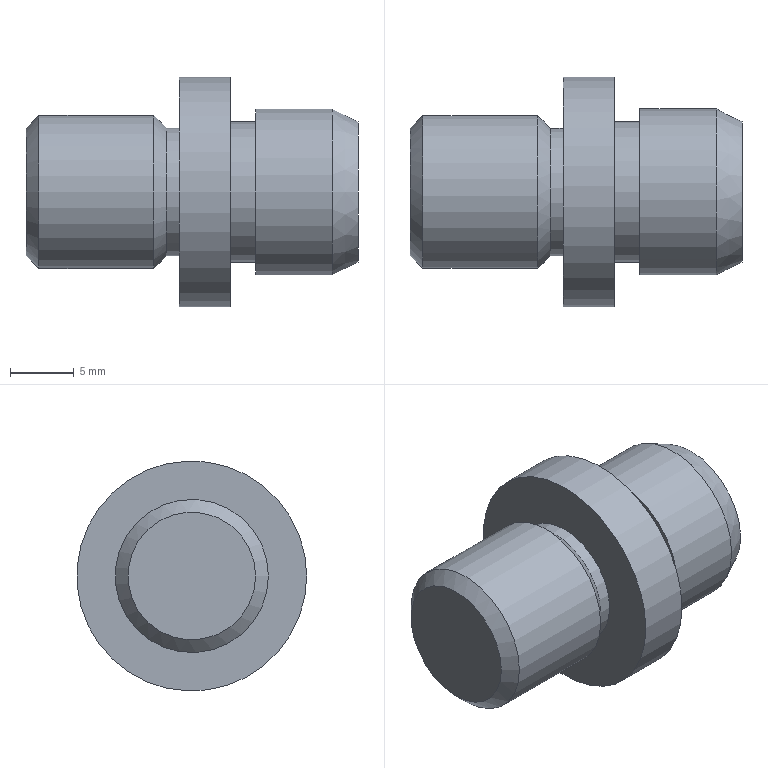Component | NX | LOC_PIN | 1 solid | 13 faces | box 26 x 18 x 18 mm | volume 3518 mm3 | plane 5 | cylinder 5 | cone 3 | commonest cylinder face diameters 12 x1 10 x1 18 x1 11 x1 13 x1
STEP:
#1=CARTESIAN_POINT('',(0.,0.,0.));
#2=DIRECTION('',(0.,0.,1.));
#3=DIRECTION('',(1.,0.,0.));
#4=AXIS2_PLACEMENT_3D('',#1,#2,#3);
#5=CARTESIAN_POINT('',(6.,75.339,-338.901));
#6=VERTEX_POINT('',#5);
#7=CARTESIAN_POINT('',(6.,80.839,-338.901));
#8=DIRECTION('',(-1.,-0.,0.));
#9=DIRECTION('',(0.,-1.,0.));
#10=AXIS2_PLACEMENT_3D('',#7,#8,#9);
#11=CIRCLE('',#10,5.5);
#12=CARTESIAN_POINT('',(6.,80.839,-338.901));
#13=DIRECTION('',(-1.,-0.,0.));
#14=DIRECTION('',(0.,-1.,0.));
#15=AXIS2_PLACEMENT_3D('',#12,#13,#14);
#16=PLANE('',#15);
#17=CARTESIAN_POINT('',(0.,0.));
#18=DIRECTION('',(1.,0.));
#19=AXIS2_PLACEMENT_2D('',#17,#18);
#20=CIRCLE('',#19,5.5);
#21=(GEOMETRIC_REPRESENTATION_CONTEXT(2)PARAMETRIC_REPRESENTATION_CONTEXT()REPRESENTATION_CONTEXT('',''));
#22=DEFINITIONAL_REPRESENTATION('',(#20),#21);
#23=PCURVE('',#16,#22);
#24=CARTESIAN_POINT('',(6.,80.839,-338.901));
#25=DIRECTION('',(-1.,-0.,0.));
#26=DIRECTION('',(0.,-1.,0.));
#27=AXIS2_PLACEMENT_3D('',#24,#25,#26);
#28=CONICAL_SURFACE('',#27,5.5,0.4636);
#29=CARTESIAN_POINT('',(0.,0.));
#30=DIRECTION('',(1.,0.));
#31=VECTOR('',#30,1.);
#32=LINE('',#29,#31);
#33=(GEOMETRIC_REPRESENTATION_CONTEXT(2)PARAMETRIC_REPRESENTATION_CONTEXT()REPRESENTATION_CONTEXT('',''));
#34=DEFINITIONAL_REPRESENTATION('',(#32),#33);
#35=PCURVE('',#28,#34);
#36=SURFACE_CURVE('',#11,(#23,#35),.PCURVE_S1.);
#37=EDGE_CURVE('',#6,#6,#36,.T.);
#38=ORIENTED_EDGE('',*,*,#37,.F.);
#39=EDGE_LOOP('',(#38));
#40=FACE_BOUND('',#39,.T.);
#41=ADVANCED_FACE('',(#40),#16,.F.);
#42=CARTESIAN_POINT('',(-20.,75.839,-338.901));
#43=VERTEX_POINT('',#42);
#44=CARTESIAN_POINT('',(-20.,80.839,-338.901));
#45=DIRECTION('',(-1.,-0.,0.));
#46=DIRECTION('',(0.,-1.,0.));
#47=AXIS2_PLACEMENT_3D('',#44,#45,#46);
#48=CIRCLE('',#47,5.);
#49=CARTESIAN_POINT('',(-20.,80.839,-338.901));
#50=DIRECTION('',(-1.,-0.,0.));
#51=DIRECTION('',(0.,-1.,0.));
#52=AXIS2_PLACEMENT_3D('',#49,#50,#51);
#53=PLANE('',#52);
#54=CARTESIAN_POINT('',(0.,0.));
#55=DIRECTION('',(1.,0.));
#56=AXIS2_PLACEMENT_2D('',#54,#55);
#57=CIRCLE('',#56,5.);
#58=(GEOMETRIC_REPRESENTATION_CONTEXT(2)PARAMETRIC_REPRESENTATION_CONTEXT()REPRESENTATION_CONTEXT('',''));
#59=DEFINITIONAL_REPRESENTATION('',(#57),#58);
#60=PCURVE('',#53,#59);
#61=CARTESIAN_POINT('',(-19.,80.839,-338.901));
#62=DIRECTION('',(1.,0.,0.));
#63=DIRECTION('',(-0.,1.,0.));
#64=AXIS2_PLACEMENT_3D('',#61,#62,#63);
#65=CONICAL_SURFACE('',#64,6.,0.7854);
#66=CARTESIAN_POINT('',(9.425,-1.));
#67=DIRECTION('',(-1.,0.));
#68=VECTOR('',#67,1.);
#69=LINE('',#66,#68);
#70=(GEOMETRIC_REPRESENTATION_CONTEXT(2)PARAMETRIC_REPRESENTATION_CONTEXT()REPRESENTATION_CONTEXT('',''));
#71=DEFINITIONAL_REPRESENTATION('',(#69),#70);
#72=PCURVE('',#65,#71);
#73=SURFACE_CURVE('',#48,(#60,#72),.PCURVE_S1.);
#74=EDGE_CURVE('',#43,#43,#73,.T.);
#75=ORIENTED_EDGE('',*,*,#74,.T.);
#76=EDGE_LOOP('',(#75));
#77=FACE_BOUND('',#76,.T.);
#78=ADVANCED_FACE('',(#77),#53,.T.);
#79=ORIENTED_EDGE('',*,*,#74,.F.);
#80=CARTESIAN_POINT('',(-19.,74.839,-338.901));
#81=VERTEX_POINT('',#80);
#82=CARTESIAN_POINT('',(-20.,75.839,-338.901));
#83=CARTESIAN_POINT('',(-19.,74.839,-338.901));
#84=B_SPLINE_CURVE_WITH_KNOTS('',1,(#82,#83),.UNSPECIFIED.,.F.,.F.,(2,2),(-1.414,-0.),.PIECEWISE_BEZIER_KNOTS.);
#85=CARTESIAN_POINT('',(9.425,0.));
#86=DIRECTION('',(0.,1.));
#87=VECTOR('',#86,1.);
#88=LINE('',#85,#87);
#89=(GEOMETRIC_REPRESENTATION_CONTEXT(2)PARAMETRIC_REPRESENTATION_CONTEXT()REPRESENTATION_CONTEXT('',''));
#90=DEFINITIONAL_REPRESENTATION('',(#88),#89);
#91=PCURVE('',#65,#90);
#92=CARTESIAN_POINT('',(3.142,0.));
#93=DIRECTION('',(0.,1.));
#94=VECTOR('',#93,1.);
#95=LINE('',#92,#94);
#96=(GEOMETRIC_REPRESENTATION_CONTEXT(2)PARAMETRIC_REPRESENTATION_CONTEXT()REPRESENTATION_CONTEXT('',''));
#97=DEFINITIONAL_REPRESENTATION('',(#95),#96);
#98=PCURVE('',#65,#97);
#99=SEAM_CURVE('',#84,(#91,#98),.PCURVE_S1.);
#100=EDGE_CURVE('',#43,#81,#99,.T.);
#101=ORIENTED_EDGE('',*,*,#100,.T.);
#102=CARTESIAN_POINT('',(-19.,80.839,-338.901));
#103=DIRECTION('',(-1.,-0.,0.));
#104=DIRECTION('',(0.,-1.,0.));
#105=AXIS2_PLACEMENT_3D('',#102,#103,#104);
#106=CIRCLE('',#105,6.);
#107=CARTESIAN_POINT('',(9.425,-0.));
#108=DIRECTION('',(-1.,0.));
#109=VECTOR('',#108,1.);
#110=LINE('',#107,#109);
#111=(GEOMETRIC_REPRESENTATION_CONTEXT(2)PARAMETRIC_REPRESENTATION_CONTEXT()REPRESENTATION_CONTEXT('',''));
#112=DEFINITIONAL_REPRESENTATION('',(#110),#111);
#113=PCURVE('',#65,#112);
#114=CARTESIAN_POINT('',(-28.,80.839,-338.901));
#115=DIRECTION('',(-1.,-0.,0.));
#116=DIRECTION('',(0.,-1.,0.));
#117=AXIS2_PLACEMENT_3D('',#114,#115,#116);
#118=CYLINDRICAL_SURFACE('',#117,6.);
#119=CARTESIAN_POINT('',(0.,-9.));
#120=DIRECTION('',(1.,0.));
#121=VECTOR('',#120,1.);
#122=LINE('',#119,#121);
#123=(GEOMETRIC_REPRESENTATION_CONTEXT(2)PARAMETRIC_REPRESENTATION_CONTEXT()REPRESENTATION_CONTEXT('',''));
#124=DEFINITIONAL_REPRESENTATION('',(#122),#123);
#125=PCURVE('',#118,#124);
#126=SURFACE_CURVE('',#106,(#113,#125),.PCURVE_S1.);
#127=EDGE_CURVE('',#81,#81,#126,.T.);
#128=ORIENTED_EDGE('',*,*,#127,.T.);
#129=ORIENTED_EDGE('',*,*,#100,.F.);
#130=EDGE_LOOP('',(#79,#101,#128,#129));
#131=FACE_BOUND('',#130,.T.);
#132=ADVANCED_FACE('',(#131),#65,.T.);
#133=ORIENTED_EDGE('',*,*,#127,.F.);
#134=CARTESIAN_POINT('',(-10.,74.839,-338.901));
#135=VERTEX_POINT('',#134);
#136=CARTESIAN_POINT('',(-10.,74.839,-338.901));
#137=CARTESIAN_POINT('',(-19.,74.839,-338.901));
#138=B_SPLINE_CURVE_WITH_KNOTS('',1,(#136,#137),.UNSPECIFIED.,.F.,.F.,(2,2),(-18.,-9.),.PIECEWISE_BEZIER_KNOTS.);
#139=CARTESIAN_POINT('',(0.,0.));
#140=DIRECTION('',(0.,1.));
#141=VECTOR('',#140,1.);
#142=LINE('',#139,#141);
#143=(GEOMETRIC_REPRESENTATION_CONTEXT(2)PARAMETRIC_REPRESENTATION_CONTEXT()REPRESENTATION_CONTEXT('',''));
#144=DEFINITIONAL_REPRESENTATION('',(#142),#143);
#145=PCURVE('',#118,#144);
#146=CARTESIAN_POINT('',(6.283,0.));
#147=DIRECTION('',(0.,1.));
#148=VECTOR('',#147,1.);
#149=LINE('',#146,#148);
#150=(GEOMETRIC_REPRESENTATION_CONTEXT(2)PARAMETRIC_REPRESENTATION_CONTEXT()REPRESENTATION_CONTEXT('',''));
#151=DEFINITIONAL_REPRESENTATION('',(#149),#150);
#152=PCURVE('',#118,#151);
#153=SEAM_CURVE('',#138,(#145,#152),.PCURVE_S1.);
#154=EDGE_CURVE('',#135,#81,#153,.T.);
#155=ORIENTED_EDGE('',*,*,#154,.F.);
#156=CARTESIAN_POINT('',(-10.,80.839,-338.901));
#157=DIRECTION('',(-1.,-0.,0.));
#158=DIRECTION('',(0.,-1.,0.));
#159=AXIS2_PLACEMENT_3D('',#156,#157,#158);
#160=CIRCLE('',#159,6.);
#161=CARTESIAN_POINT('',(0.,-18.));
#162=DIRECTION('',(1.,0.));
#163=VECTOR('',#162,1.);
#164=LINE('',#161,#163);
#165=(GEOMETRIC_REPRESENTATION_CONTEXT(2)PARAMETRIC_REPRESENTATION_CONTEXT()REPRESENTATION_CONTEXT('',''));
#166=DEFINITIONAL_REPRESENTATION('',(#164),#165);
#167=PCURVE('',#118,#166);
#168=CARTESIAN_POINT('',(-9.,80.839,-338.901));
#169=DIRECTION('',(-1.,-0.,0.));
#170=DIRECTION('',(0.,-1.,0.));
#171=AXIS2_PLACEMENT_3D('',#168,#169,#170);
#172=CONICAL_SURFACE('',#171,5.,0.7854);
#173=CARTESIAN_POINT('',(0.,1.));
#174=DIRECTION('',(1.,0.));
#175=VECTOR('',#174,1.);
#176=LINE('',#173,#175);
#177=(GEOMETRIC_REPRESENTATION_CONTEXT(2)PARAMETRIC_REPRESENTATION_CONTEXT()REPRESENTATION_CONTEXT('',''));
#178=DEFINITIONAL_REPRESENTATION('',(#176),#177);
#179=PCURVE('',#172,#178);
#180=SURFACE_CURVE('',#160,(#167,#179),.PCURVE_S1.);
#181=EDGE_CURVE('',#135,#135,#180,.T.);
#182=ORIENTED_EDGE('',*,*,#181,.T.);
#183=ORIENTED_EDGE('',*,*,#154,.T.);
#184=EDGE_LOOP('',(#133,#155,#182,#183));
#185=FACE_BOUND('',#184,.T.);
#186=ADVANCED_FACE('',(#185),#118,.T.);
#187=ORIENTED_EDGE('',*,*,#181,.F.);
#188=CARTESIAN_POINT('',(-9.,75.839,-338.901));
#189=VERTEX_POINT('',#188);
#190=CARTESIAN_POINT('',(-9.,75.839,-338.901));
#191=CARTESIAN_POINT('',(-10.,74.839,-338.901));
#192=B_SPLINE_CURVE_WITH_KNOTS('',1,(#190,#191),.UNSPECIFIED.,.F.,.F.,(2,2),(0.,1.414),.PIECEWISE_BEZIER_KNOTS.);
#193=CARTESIAN_POINT('',(0.,0.));
#194=DIRECTION('',(0.,1.));
#195=VECTOR('',#194,1.);
#196=LINE('',#193,#195);
#197=(GEOMETRIC_REPRESENTATION_CONTEXT(2)PARAMETRIC_REPRESENTATION_CONTEXT()REPRESENTATION_CONTEXT('',''));
#198=DEFINITIONAL_REPRESENTATION('',(#196),#197);
#199=PCURVE('',#172,#198);
#200=CARTESIAN_POINT('',(6.283,0.));
#201=DIRECTION('',(0.,1.));
#202=VECTOR('',#201,1.);
#203=LINE('',#200,#202);
#204=(GEOMETRIC_REPRESENTATION_CONTEXT(2)PARAMETRIC_REPRESENTATION_CONTEXT()REPRESENTATION_CONTEXT('',''));
#205=DEFINITIONAL_REPRESENTATION('',(#203),#204);
#206=PCURVE('',#172,#205);
#207=SEAM_CURVE('',#192,(#199,#206),.PCURVE_S1.);
#208=EDGE_CURVE('',#189,#135,#207,.T.);
#209=ORIENTED_EDGE('',*,*,#208,.F.);
#210=CARTESIAN_POINT('',(-9.,80.839,-338.901));
#211=DIRECTION('',(-1.,-0.,0.));
#212=DIRECTION('',(0.,-1.,0.));
#213=AXIS2_PLACEMENT_3D('',#210,#211,#212);
#214=CIRCLE('',#213,5.);
#215=CARTESIAN_POINT('',(0.,0.));
#216=DIRECTION('',(1.,0.));
#217=VECTOR('',#216,1.);
#218=LINE('',#215,#217);
#219=(GEOMETRIC_REPRESENTATION_CONTEXT(2)PARAMETRIC_REPRESENTATION_CONTEXT()REPRESENTATION_CONTEXT('',''));
#220=DEFINITIONAL_REPRESENTATION('',(#218),#219);
#221=PCURVE('',#172,#220);
#222=CARTESIAN_POINT('',(-28.,80.839,-338.901));
#223=DIRECTION('',(-1.,-0.,0.));
#224=DIRECTION('',(0.,-1.,0.));
#225=AXIS2_PLACEMENT_3D('',#222,#223,#224);
#226=CYLINDRICAL_SURFACE('',#225,5.);
#227=CARTESIAN_POINT('',(0.,-19.));
#228=DIRECTION('',(1.,0.));
#229=VECTOR('',#228,1.);
#230=LINE('',#227,#229);
#231=(GEOMETRIC_REPRESENTATION_CONTEXT(2)PARAMETRIC_REPRESENTATION_CONTEXT()REPRESENTATION_CONTEXT('',''));
#232=DEFINITIONAL_REPRESENTATION('',(#230),#231);
#233=PCURVE('',#226,#232);
#234=SURFACE_CURVE('',#214,(#221,#233),.PCURVE_S1.);
#235=EDGE_CURVE('',#189,#189,#234,.T.);
#236=ORIENTED_EDGE('',*,*,#235,.T.);
#237=ORIENTED_EDGE('',*,*,#208,.T.);
#238=EDGE_LOOP('',(#187,#209,#236,#237));
#239=FACE_BOUND('',#238,.T.);
#240=ADVANCED_FACE('',(#239),#172,.T.);
#241=ORIENTED_EDGE('',*,*,#235,.F.);
#242=CARTESIAN_POINT('',(-8.,75.839,-338.901));
#243=VERTEX_POINT('',#242);
#244=CARTESIAN_POINT('',(-8.,75.839,-338.901));
#245=CARTESIAN_POINT('',(-9.,75.839,-338.901));
#246=B_SPLINE_CURVE_WITH_KNOTS('',1,(#244,#245),.UNSPECIFIED.,.F.,.F.,(2,2),(-20.,-19.),.PIECEWISE_BEZIER_KNOTS.);
#247=CARTESIAN_POINT('',(0.,0.));
#248=DIRECTION('',(0.,1.));
#249=VECTOR('',#248,1.);
#250=LINE('',#247,#249);
#251=(GEOMETRIC_REPRESENTATION_CONTEXT(2)PARAMETRIC_REPRESENTATION_CONTEXT()REPRESENTATION_CONTEXT('',''));
#252=DEFINITIONAL_REPRESENTATION('',(#250),#251);
#253=PCURVE('',#226,#252);
#254=CARTESIAN_POINT('',(6.283,0.));
#255=DIRECTION('',(0.,1.));
#256=VECTOR('',#255,1.);
#257=LINE('',#254,#256);
#258=(GEOMETRIC_REPRESENTATION_CONTEXT(2)PARAMETRIC_REPRESENTATION_CONTEXT()REPRESENTATION_CONTEXT('',''));
#259=DEFINITIONAL_REPRESENTATION('',(#257),#258);
#260=PCURVE('',#226,#259);
#261=SEAM_CURVE('',#246,(#253,#260),.PCURVE_S1.);
#262=EDGE_CURVE('',#243,#189,#261,.T.);
#263=ORIENTED_EDGE('',*,*,#262,.F.);
#264=CARTESIAN_POINT('',(-8.,80.839,-338.901));
#265=DIRECTION('',(-1.,-0.,0.));
#266=DIRECTION('',(0.,-1.,0.));
#267=AXIS2_PLACEMENT_3D('',#264,#265,#266);
#268=CIRCLE('',#267,5.);
#269=CARTESIAN_POINT('',(0.,-20.));
#270=DIRECTION('',(1.,0.));
#271=VECTOR('',#270,1.);
#272=LINE('',#269,#271);
#273=(GEOMETRIC_REPRESENTATION_CONTEXT(2)PARAMETRIC_REPRESENTATION_CONTEXT()REPRESENTATION_CONTEXT('',''));
#274=DEFINITIONAL_REPRESENTATION('',(#272),#273);
#275=PCURVE('',#226,#274);
#276=CARTESIAN_POINT('',(-8.,71.839,-338.901));
#277=DIRECTION('',(1.,0.,0.));
#278=DIRECTION('',(-0.,1.,0.));
#279=AXIS2_PLACEMENT_3D('',#276,#277,#278);
#280=PLANE('',#279);
#281=CARTESIAN_POINT('',(4.,0.));
#282=CARTESIAN_POINT('',(4.,8.66));
#283=CARTESIAN_POINT('',(11.5,4.33));
#284=CARTESIAN_POINT('',(19.,0.));
#285=CARTESIAN_POINT('',(11.5,-4.33));
#286=CARTESIAN_POINT('',(4.,-8.66));
#287=CARTESIAN_POINT('',(4.,0.));
#288=(BOUNDED_CURVE()B_SPLINE_CURVE(2,(#281,#282,#283,#284,#285,#286,#287),.UNSPECIFIED.,.T.,.F.)B_SPLINE_CURVE_WITH_KNOTS((1,2,2,2,2,1),(-2.094,0.,2.094,4.189,6.283,8.378),.UNSPECIFIED.)CURVE()GEOMETRIC_REPRESENTATION_ITEM()RATIONAL_B_SPLINE_CURVE((1.,0.5,1.,0.5,1.,0.5,1.))REPRESENTATION_ITEM(''));
#289=(GEOMETRIC_REPRESENTATION_CONTEXT(2)PARAMETRIC_REPRESENTATION_CONTEXT()REPRESENTATION_CONTEXT('',''));
#290=DEFINITIONAL_REPRESENTATION('',(#288),#289);
#291=PCURVE('',#280,#290);
#292=SURFACE_CURVE('',#268,(#275,#291),.PCURVE_S1.);
#293=EDGE_CURVE('',#243,#243,#292,.T.);
#294=ORIENTED_EDGE('',*,*,#293,.T.);
#295=ORIENTED_EDGE('',*,*,#262,.T.);
#296=EDGE_LOOP('',(#241,#263,#294,#295));
#297=FACE_BOUND('',#296,.T.);
#298=ADVANCED_FACE('',(#297),#226,.T.);
#299=ORIENTED_EDGE('',*,*,#293,.F.);
#300=EDGE_LOOP('',(#299));
#301=FACE_BOUND('',#300,.T.);
#302=CARTESIAN_POINT('',(-8.,71.839,-338.901));
#303=VERTEX_POINT('',#302);
#304=CARTESIAN_POINT('',(-8.,80.839,-338.901));
#305=DIRECTION('',(-1.,-0.,0.));
#306=DIRECTION('',(0.,-1.,0.));
#307=AXIS2_PLACEMENT_3D('',#304,#305,#306);
#308=CIRCLE('',#307,9.);
#309=CARTESIAN_POINT('',(0.,0.));
#310=CARTESIAN_POINT('',(0.,15.588));
#311=CARTESIAN_POINT('',(13.5,7.794));
#312=CARTESIAN_POINT('',(27.,0.));
#313=CARTESIAN_POINT('',(13.5,-7.794));
#314=CARTESIAN_POINT('',(0.,-15.588));
#315=CARTESIAN_POINT('',(0.,0.));
#316=(BOUNDED_CURVE()B_SPLINE_CURVE(2,(#309,#310,#311,#312,#313,#314,#315),.UNSPECIFIED.,.T.,.F.)B_SPLINE_CURVE_WITH_KNOTS((1,2,2,2,2,1),(-2.094,0.,2.094,4.189,6.283,8.378),.UNSPECIFIED.)CURVE()GEOMETRIC_REPRESENTATION_ITEM()RATIONAL_B_SPLINE_CURVE((1.,0.5,1.,0.5,1.,0.5,1.))REPRESENTATION_ITEM(''));
#317=(GEOMETRIC_REPRESENTATION_CONTEXT(2)PARAMETRIC_REPRESENTATION_CONTEXT()REPRESENTATION_CONTEXT('',''));
#318=DEFINITIONAL_REPRESENTATION('',(#316),#317);
#319=PCURVE('',#280,#318);
#320=CARTESIAN_POINT('',(-28.,80.839,-338.901));
#321=DIRECTION('',(-1.,-0.,0.));
#322=DIRECTION('',(0.,-1.,0.));
#323=AXIS2_PLACEMENT_3D('',#320,#321,#322);
#324=CYLINDRICAL_SURFACE('',#323,9.);
#325=CARTESIAN_POINT('',(0.,-20.));
#326=DIRECTION('',(1.,0.));
#327=VECTOR('',#326,1.);
#328=LINE('',#325,#327);
#329=(GEOMETRIC_REPRESENTATION_CONTEXT(2)PARAMETRIC_REPRESENTATION_CONTEXT()REPRESENTATION_CONTEXT('',''));
#330=DEFINITIONAL_REPRESENTATION('',(#328),#329);
#331=PCURVE('',#324,#330);
#332=SURFACE_CURVE('',#308,(#319,#331),.PCURVE_S1.);
#333=EDGE_CURVE('',#303,#303,#332,.T.);
#334=ORIENTED_EDGE('',*,*,#333,.T.);
#335=EDGE_LOOP('',(#334));
#336=FACE_BOUND('',#335,.T.);
#337=ADVANCED_FACE('',(#301,#336),#280,.F.);
#338=ORIENTED_EDGE('',*,*,#333,.F.);
#339=CARTESIAN_POINT('',(-4.,71.839,-338.901));
#340=VERTEX_POINT('',#339);
#341=CARTESIAN_POINT('',(-4.,71.839,-338.901));
#342=CARTESIAN_POINT('',(-8.,71.839,-338.901));
#343=B_SPLINE_CURVE_WITH_KNOTS('',1,(#341,#342),.UNSPECIFIED.,.F.,.F.,(2,2),(-24.,-20.),.PIECEWISE_BEZIER_KNOTS.);
#344=CARTESIAN_POINT('',(0.,0.));
#345=DIRECTION('',(0.,1.));
#346=VECTOR('',#345,1.);
#347=LINE('',#344,#346);
#348=(GEOMETRIC_REPRESENTATION_CONTEXT(2)PARAMETRIC_REPRESENTATION_CONTEXT()REPRESENTATION_CONTEXT('',''));
#349=DEFINITIONAL_REPRESENTATION('',(#347),#348);
#350=PCURVE('',#324,#349);
#351=CARTESIAN_POINT('',(6.283,0.));
#352=DIRECTION('',(0.,1.));
#353=VECTOR('',#352,1.);
#354=LINE('',#351,#353);
#355=(GEOMETRIC_REPRESENTATION_CONTEXT(2)PARAMETRIC_REPRESENTATION_CONTEXT()REPRESENTATION_CONTEXT('',''));
#356=DEFINITIONAL_REPRESENTATION('',(#354),#355);
#357=PCURVE('',#324,#356);
#358=SEAM_CURVE('',#343,(#350,#357),.PCURVE_S1.);
#359=EDGE_CURVE('',#340,#303,#358,.T.);
#360=ORIENTED_EDGE('',*,*,#359,.F.);
#361=CARTESIAN_POINT('',(-4.,80.839,-338.901));
#362=DIRECTION('',(-1.,-0.,0.));
#363=DIRECTION('',(0.,-1.,0.));
#364=AXIS2_PLACEMENT_3D('',#361,#362,#363);
#365=CIRCLE('',#364,9.);
#366=CARTESIAN_POINT('',(0.,-24.));
#367=DIRECTION('',(1.,0.));
#368=VECTOR('',#367,1.);
#369=LINE('',#366,#368);
#370=(GEOMETRIC_REPRESENTATION_CONTEXT(2)PARAMETRIC_REPRESENTATION_CONTEXT()REPRESENTATION_CONTEXT('',''));
#371=DEFINITIONAL_REPRESENTATION('',(#369),#370);
#372=PCURVE('',#324,#371);
#373=CARTESIAN_POINT('',(-4.,75.339,-338.901));
#374=DIRECTION('',(-1.,-0.,0.));
#375=DIRECTION('',(0.,-1.,0.));
#376=AXIS2_PLACEMENT_3D('',#373,#374,#375);
#377=PLANE('',#376);
#378=CARTESIAN_POINT('',(-5.5,0.));
#379=DIRECTION('',(1.,0.));
#380=AXIS2_PLACEMENT_2D('',#378,#379);
#381=CIRCLE('',#380,9.);
#382=(GEOMETRIC_REPRESENTATION_CONTEXT(2)PARAMETRIC_REPRESENTATION_CONTEXT()REPRESENTATION_CONTEXT('',''));
#383=DEFINITIONAL_REPRESENTATION('',(#381),#382);
#384=PCURVE('',#377,#383);
#385=SURFACE_CURVE('',#365,(#372,#384),.PCURVE_S1.);
#386=EDGE_CURVE('',#340,#340,#385,.T.);
#387=ORIENTED_EDGE('',*,*,#386,.T.);
#388=ORIENTED_EDGE('',*,*,#359,.T.);
#389=EDGE_LOOP('',(#338,#360,#387,#388));
#390=FACE_BOUND('',#389,.T.);
#391=ADVANCED_FACE('',(#390),#324,.T.);
#392=ORIENTED_EDGE('',*,*,#386,.F.);
#393=EDGE_LOOP('',(#392));
#394=FACE_BOUND('',#393,.T.);
#395=CARTESIAN_POINT('',(-4.,75.339,-338.901));
#396=VERTEX_POINT('',#395);
#397=CARTESIAN_POINT('',(-4.,80.839,-338.901));
#398=DIRECTION('',(-1.,-0.,0.));
#399=DIRECTION('',(0.,-1.,0.));
#400=AXIS2_PLACEMENT_3D('',#397,#398,#399);
#401=CIRCLE('',#400,5.5);
#402=CARTESIAN_POINT('',(-5.5,0.));
#403=DIRECTION('',(1.,0.));
#404=AXIS2_PLACEMENT_2D('',#402,#403);
#405=CIRCLE('',#404,5.5);
#406=(GEOMETRIC_REPRESENTATION_CONTEXT(2)PARAMETRIC_REPRESENTATION_CONTEXT()REPRESENTATION_CONTEXT('',''));
#407=DEFINITIONAL_REPRESENTATION('',(#405),#406);
#408=PCURVE('',#377,#407);
#409=CARTESIAN_POINT('',(-28.,80.839,-338.901));
#410=DIRECTION('',(-1.,-0.,0.));
#411=DIRECTION('',(0.,-1.,0.));
#412=AXIS2_PLACEMENT_3D('',#409,#410,#411);
#413=CYLINDRICAL_SURFACE('',#412,5.5);
#414=CARTESIAN_POINT('',(0.,-24.));
#415=DIRECTION('',(1.,0.));
#416=VECTOR('',#415,1.);
#417=LINE('',#414,#416);
#418=(GEOMETRIC_REPRESENTATION_CONTEXT(2)PARAMETRIC_REPRESENTATION_CONTEXT()REPRESENTATION_CONTEXT('',''));
#419=DEFINITIONAL_REPRESENTATION('',(#417),#418);
#420=PCURVE('',#413,#419);
#421=SURFACE_CURVE('',#401,(#408,#420),.PCURVE_S1.);
#422=EDGE_CURVE('',#396,#396,#421,.T.);
#423=ORIENTED_EDGE('',*,*,#422,.T.);
#424=EDGE_LOOP('',(#423));
#425=FACE_BOUND('',#424,.T.);
#426=ADVANCED_FACE('',(#394,#425),#377,.F.);
#427=ORIENTED_EDGE('',*,*,#422,.F.);
#428=CARTESIAN_POINT('',(-2.,75.339,-338.901));
#429=VERTEX_POINT('',#428);
#430=CARTESIAN_POINT('',(-2.,75.339,-338.901));
#431=CARTESIAN_POINT('',(-4.,75.339,-338.901));
#432=B_SPLINE_CURVE_WITH_KNOTS('',1,(#430,#431),.UNSPECIFIED.,.F.,.F.,(2,2),(-26.,-24.),.PIECEWISE_BEZIER_KNOTS.);
#433=CARTESIAN_POINT('',(0.,0.));
#434=DIRECTION('',(0.,1.));
#435=VECTOR('',#434,1.);
#436=LINE('',#433,#435);
#437=(GEOMETRIC_REPRESENTATION_CONTEXT(2)PARAMETRIC_REPRESENTATION_CONTEXT()REPRESENTATION_CONTEXT('',''));
#438=DEFINITIONAL_REPRESENTATION('',(#436),#437);
#439=PCURVE('',#413,#438);
#440=CARTESIAN_POINT('',(6.283,0.));
#441=DIRECTION('',(0.,1.));
#442=VECTOR('',#441,1.);
#443=LINE('',#440,#442);
#444=(GEOMETRIC_REPRESENTATION_CONTEXT(2)PARAMETRIC_REPRESENTATION_CONTEXT()REPRESENTATION_CONTEXT('',''));
#445=DEFINITIONAL_REPRESENTATION('',(#443),#444);
#446=PCURVE('',#413,#445);
#447=SEAM_CURVE('',#432,(#439,#446),.PCURVE_S1.);
#448=EDGE_CURVE('',#429,#396,#447,.T.);
#449=ORIENTED_EDGE('',*,*,#448,.F.);
#450=CARTESIAN_POINT('',(-2.,80.839,-338.901));
#451=DIRECTION('',(-1.,-0.,0.));
#452=DIRECTION('',(0.,-1.,0.));
#453=AXIS2_PLACEMENT_3D('',#450,#451,#452);
#454=CIRCLE('',#453,5.5);
#455=CARTESIAN_POINT('',(0.,-26.));
#456=DIRECTION('',(1.,0.));
#457=VECTOR('',#456,1.);
#458=LINE('',#455,#457);
#459=(GEOMETRIC_REPRESENTATION_CONTEXT(2)PARAMETRIC_REPRESENTATION_CONTEXT()REPRESENTATION_CONTEXT('',''));
#460=DEFINITIONAL_REPRESENTATION('',(#458),#459);
#461=PCURVE('',#413,#460);
#462=CARTESIAN_POINT('',(-2.,74.339,-338.901));
#463=DIRECTION('',(1.,0.,0.));
#464=DIRECTION('',(-0.,1.,0.));
#465=AXIS2_PLACEMENT_3D('',#462,#463,#464);
#466=PLANE('',#465);
#467=CARTESIAN_POINT('',(1.,0.));
#468=CARTESIAN_POINT('',(1.,9.526));
#469=CARTESIAN_POINT('',(9.25,4.763));
#470=CARTESIAN_POINT('',(17.5,0.));
#471=CARTESIAN_POINT('',(9.25,-4.763));
#472=CARTESIAN_POINT('',(1.,-9.526));
#473=CARTESIAN_POINT('',(1.,0.));
#474=(BOUNDED_CURVE()B_SPLINE_CURVE(2,(#467,#468,#469,#470,#471,#472,#473),.UNSPECIFIED.,.T.,.F.)B_SPLINE_CURVE_WITH_KNOTS((1,2,2,2,2,1),(-2.094,0.,2.094,4.189,6.283,8.378),.UNSPECIFIED.)CURVE()GEOMETRIC_REPRESENTATION_ITEM()RATIONAL_B_SPLINE_CURVE((1.,0.5,1.,0.5,1.,0.5,1.))REPRESENTATION_ITEM(''));
#475=(GEOMETRIC_REPRESENTATION_CONTEXT(2)PARAMETRIC_REPRESENTATION_CONTEXT()REPRESENTATION_CONTEXT('',''));
#476=DEFINITIONAL_REPRESENTATION('',(#474),#475);
#477=PCURVE('',#466,#476);
#478=SURFACE_CURVE('',#454,(#461,#477),.PCURVE_S1.);
#479=EDGE_CURVE('',#429,#429,#478,.T.);
#480=ORIENTED_EDGE('',*,*,#479,.T.);
#481=ORIENTED_EDGE('',*,*,#448,.T.);
#482=EDGE_LOOP('',(#427,#449,#480,#481));
#483=FACE_BOUND('',#482,.T.);
#484=ADVANCED_FACE('',(#483),#413,.T.);
#485=ORIENTED_EDGE('',*,*,#479,.F.);
#486=EDGE_LOOP('',(#485));
#487=FACE_BOUND('',#486,.T.);
#488=CARTESIAN_POINT('',(-2.,74.339,-338.901));
#489=VERTEX_POINT('',#488);
#490=CARTESIAN_POINT('',(-2.,80.839,-338.901));
#491=DIRECTION('',(-1.,-0.,0.));
#492=DIRECTION('',(0.,-1.,0.));
#493=AXIS2_PLACEMENT_3D('',#490,#491,#492);
#494=CIRCLE('',#493,6.5);
#495=CARTESIAN_POINT('',(0.,0.));
#496=CARTESIAN_POINT('',(0.,11.258));
#497=CARTESIAN_POINT('',(9.75,5.629));
#498=CARTESIAN_POINT('',(19.5,0.));
#499=CARTESIAN_POINT('',(9.75,-5.629));
#500=CARTESIAN_POINT('',(0.,-11.258));
#501=CARTESIAN_POINT('',(0.,0.));
#502=(BOUNDED_CURVE()B_SPLINE_CURVE(2,(#495,#496,#497,#498,#499,#500,#501),.UNSPECIFIED.,.T.,.F.)B_SPLINE_CURVE_WITH_KNOTS((1,2,2,2,2,1),(-2.094,0.,2.094,4.189,6.283,8.378),.UNSPECIFIED.)CURVE()GEOMETRIC_REPRESENTATION_ITEM()RATIONAL_B_SPLINE_CURVE((1.,0.5,1.,0.5,1.,0.5,1.))REPRESENTATION_ITEM(''));
#503=(GEOMETRIC_REPRESENTATION_CONTEXT(2)PARAMETRIC_REPRESENTATION_CONTEXT()REPRESENTATION_CONTEXT('',''));
#504=DEFINITIONAL_REPRESENTATION('',(#502),#503);
#505=PCURVE('',#466,#504);
#506=CARTESIAN_POINT('',(-28.,80.839,-338.901));
#507=DIRECTION('',(-1.,-0.,0.));
#508=DIRECTION('',(0.,-1.,0.));
#509=AXIS2_PLACEMENT_3D('',#506,#507,#508);
#510=CYLINDRICAL_SURFACE('',#509,6.5);
#511=CARTESIAN_POINT('',(0.,-26.));
#512=DIRECTION('',(1.,0.));
#513=VECTOR('',#512,1.);
#514=LINE('',#511,#513);
#515=(GEOMETRIC_REPRESENTATION_CONTEXT(2)PARAMETRIC_REPRESENTATION_CONTEXT()REPRESENTATION_CONTEXT('',''));
#516=DEFINITIONAL_REPRESENTATION('',(#514),#515);
#517=PCURVE('',#510,#516);
#518=SURFACE_CURVE('',#494,(#505,#517),.PCURVE_S1.);
#519=EDGE_CURVE('',#489,#489,#518,.T.);
#520=ORIENTED_EDGE('',*,*,#519,.T.);
#521=EDGE_LOOP('',(#520));
#522=FACE_BOUND('',#521,.T.);
#523=ADVANCED_FACE('',(#487,#522),#466,.F.);
#524=ORIENTED_EDGE('',*,*,#519,.F.);
#525=CARTESIAN_POINT('',(4.,74.339,-338.901));
#526=VERTEX_POINT('',#525);
#527=CARTESIAN_POINT('',(4.,74.339,-338.901));
#528=CARTESIAN_POINT('',(-2.,74.339,-338.901));
#529=B_SPLINE_CURVE_WITH_KNOTS('',1,(#527,#528),.UNSPECIFIED.,.F.,.F.,(2,2),(-32.,-26.),.PIECEWISE_BEZIER_KNOTS.);
#530=CARTESIAN_POINT('',(0.,0.));
#531=DIRECTION('',(0.,1.));
#532=VECTOR('',#531,1.);
#533=LINE('',#530,#532);
#534=(GEOMETRIC_REPRESENTATION_CONTEXT(2)PARAMETRIC_REPRESENTATION_CONTEXT()REPRESENTATION_CONTEXT('',''));
#535=DEFINITIONAL_REPRESENTATION('',(#533),#534);
#536=PCURVE('',#510,#535);
#537=CARTESIAN_POINT('',(6.283,0.));
#538=DIRECTION('',(0.,1.));
#539=VECTOR('',#538,1.);
#540=LINE('',#537,#539);
#541=(GEOMETRIC_REPRESENTATION_CONTEXT(2)PARAMETRIC_REPRESENTATION_CONTEXT()REPRESENTATION_CONTEXT('',''));
#542=DEFINITIONAL_REPRESENTATION('',(#540),#541);
#543=PCURVE('',#510,#542);
#544=SEAM_CURVE('',#529,(#536,#543),.PCURVE_S1.);
#545=EDGE_CURVE('',#526,#489,#544,.T.);
#546=ORIENTED_EDGE('',*,*,#545,.F.);
#547=CARTESIAN_POINT('',(4.,80.839,-338.901));
#548=DIRECTION('',(-1.,-0.,0.));
#549=DIRECTION('',(0.,-1.,0.));
#550=AXIS2_PLACEMENT_3D('',#547,#548,#549);
#551=CIRCLE('',#550,6.5);
#552=CARTESIAN_POINT('',(0.,-32.));
#553=DIRECTION('',(1.,0.));
#554=VECTOR('',#553,1.);
#555=LINE('',#552,#554);
#556=(GEOMETRIC_REPRESENTATION_CONTEXT(2)PARAMETRIC_REPRESENTATION_CONTEXT()REPRESENTATION_CONTEXT('',''));
#557=DEFINITIONAL_REPRESENTATION('',(#555),#556);
#558=PCURVE('',#510,#557);
#559=CARTESIAN_POINT('',(0.,2.));
#560=DIRECTION('',(1.,0.));
#561=VECTOR('',#560,1.);
#562=LINE('',#559,#561);
#563=(GEOMETRIC_REPRESENTATION_CONTEXT(2)PARAMETRIC_REPRESENTATION_CONTEXT()REPRESENTATION_CONTEXT('',''));
#564=DEFINITIONAL_REPRESENTATION('',(#562),#563);
#565=PCURVE('',#28,#564);
#566=SURFACE_CURVE('',#551,(#558,#565),.PCURVE_S1.);
#567=EDGE_CURVE('',#526,#526,#566,.T.);
#568=ORIENTED_EDGE('',*,*,#567,.T.);
#569=ORIENTED_EDGE('',*,*,#545,.T.);
#570=EDGE_LOOP('',(#524,#546,#568,#569));
#571=FACE_BOUND('',#570,.T.);
#572=ADVANCED_FACE('',(#571),#510,.T.);
#573=ORIENTED_EDGE('',*,*,#567,.F.);
#574=CARTESIAN_POINT('',(6.,75.339,-338.901));
#575=CARTESIAN_POINT('',(4.,74.339,-338.901));
#576=B_SPLINE_CURVE_WITH_KNOTS('',1,(#574,#575),.UNSPECIFIED.,.F.,.F.,(2,2),(0.,2.236),.PIECEWISE_BEZIER_KNOTS.);
#577=CARTESIAN_POINT('',(0.,0.));
#578=DIRECTION('',(0.,1.));
#579=VECTOR('',#578,1.);
#580=LINE('',#577,#579);
#581=(GEOMETRIC_REPRESENTATION_CONTEXT(2)PARAMETRIC_REPRESENTATION_CONTEXT()REPRESENTATION_CONTEXT('',''));
#582=DEFINITIONAL_REPRESENTATION('',(#580),#581);
#583=PCURVE('',#28,#582);
#584=CARTESIAN_POINT('',(6.283,0.));
#585=DIRECTION('',(0.,1.));
#586=VECTOR('',#585,1.);
#587=LINE('',#584,#586);
#588=(GEOMETRIC_REPRESENTATION_CONTEXT(2)PARAMETRIC_REPRESENTATION_CONTEXT()REPRESENTATION_CONTEXT('',''));
#589=DEFINITIONAL_REPRESENTATION('',(#587),#588);
#590=PCURVE('',#28,#589);
#591=SEAM_CURVE('',#576,(#583,#590),.PCURVE_S1.);
#592=EDGE_CURVE('',#6,#526,#591,.T.);
#593=ORIENTED_EDGE('',*,*,#592,.F.);
#594=ORIENTED_EDGE('',*,*,#37,.T.);
#595=ORIENTED_EDGE('',*,*,#592,.T.);
#596=EDGE_LOOP('',(#573,#593,#594,#595));
#597=FACE_BOUND('',#596,.T.);
#598=ADVANCED_FACE('',(#597),#28,.T.);
#599=CLOSED_SHELL('',(#41,#78,#132,#186,#240,#298,#337,#391,#426,#484,#523,#572,#598));
#600=MANIFOLD_SOLID_BREP('',#599);
#601=(LENGTH_UNIT()NAMED_UNIT(*)SI_UNIT(.MILLI.,.METRE.));
#602=UNCERTAINTY_MEASURE_WITH_UNIT(LENGTH_MEASURE(0.00001),#601,'','');
#603=(NAMED_UNIT(*)PLANE_ANGLE_UNIT()SI_UNIT($,.RADIAN.));
#604=(NAMED_UNIT(*)SI_UNIT($,.STERADIAN.)SOLID_ANGLE_UNIT());
#605=(GEOMETRIC_REPRESENTATION_CONTEXT(3)GLOBAL_UNCERTAINTY_ASSIGNED_CONTEXT((#602))GLOBAL_UNIT_ASSIGNED_CONTEXT((#601,#603,#604))REPRESENTATION_CONTEXT('',''));
#606=ADVANCED_BREP_SHAPE_REPRESENTATION('',(#4,#600),#605);